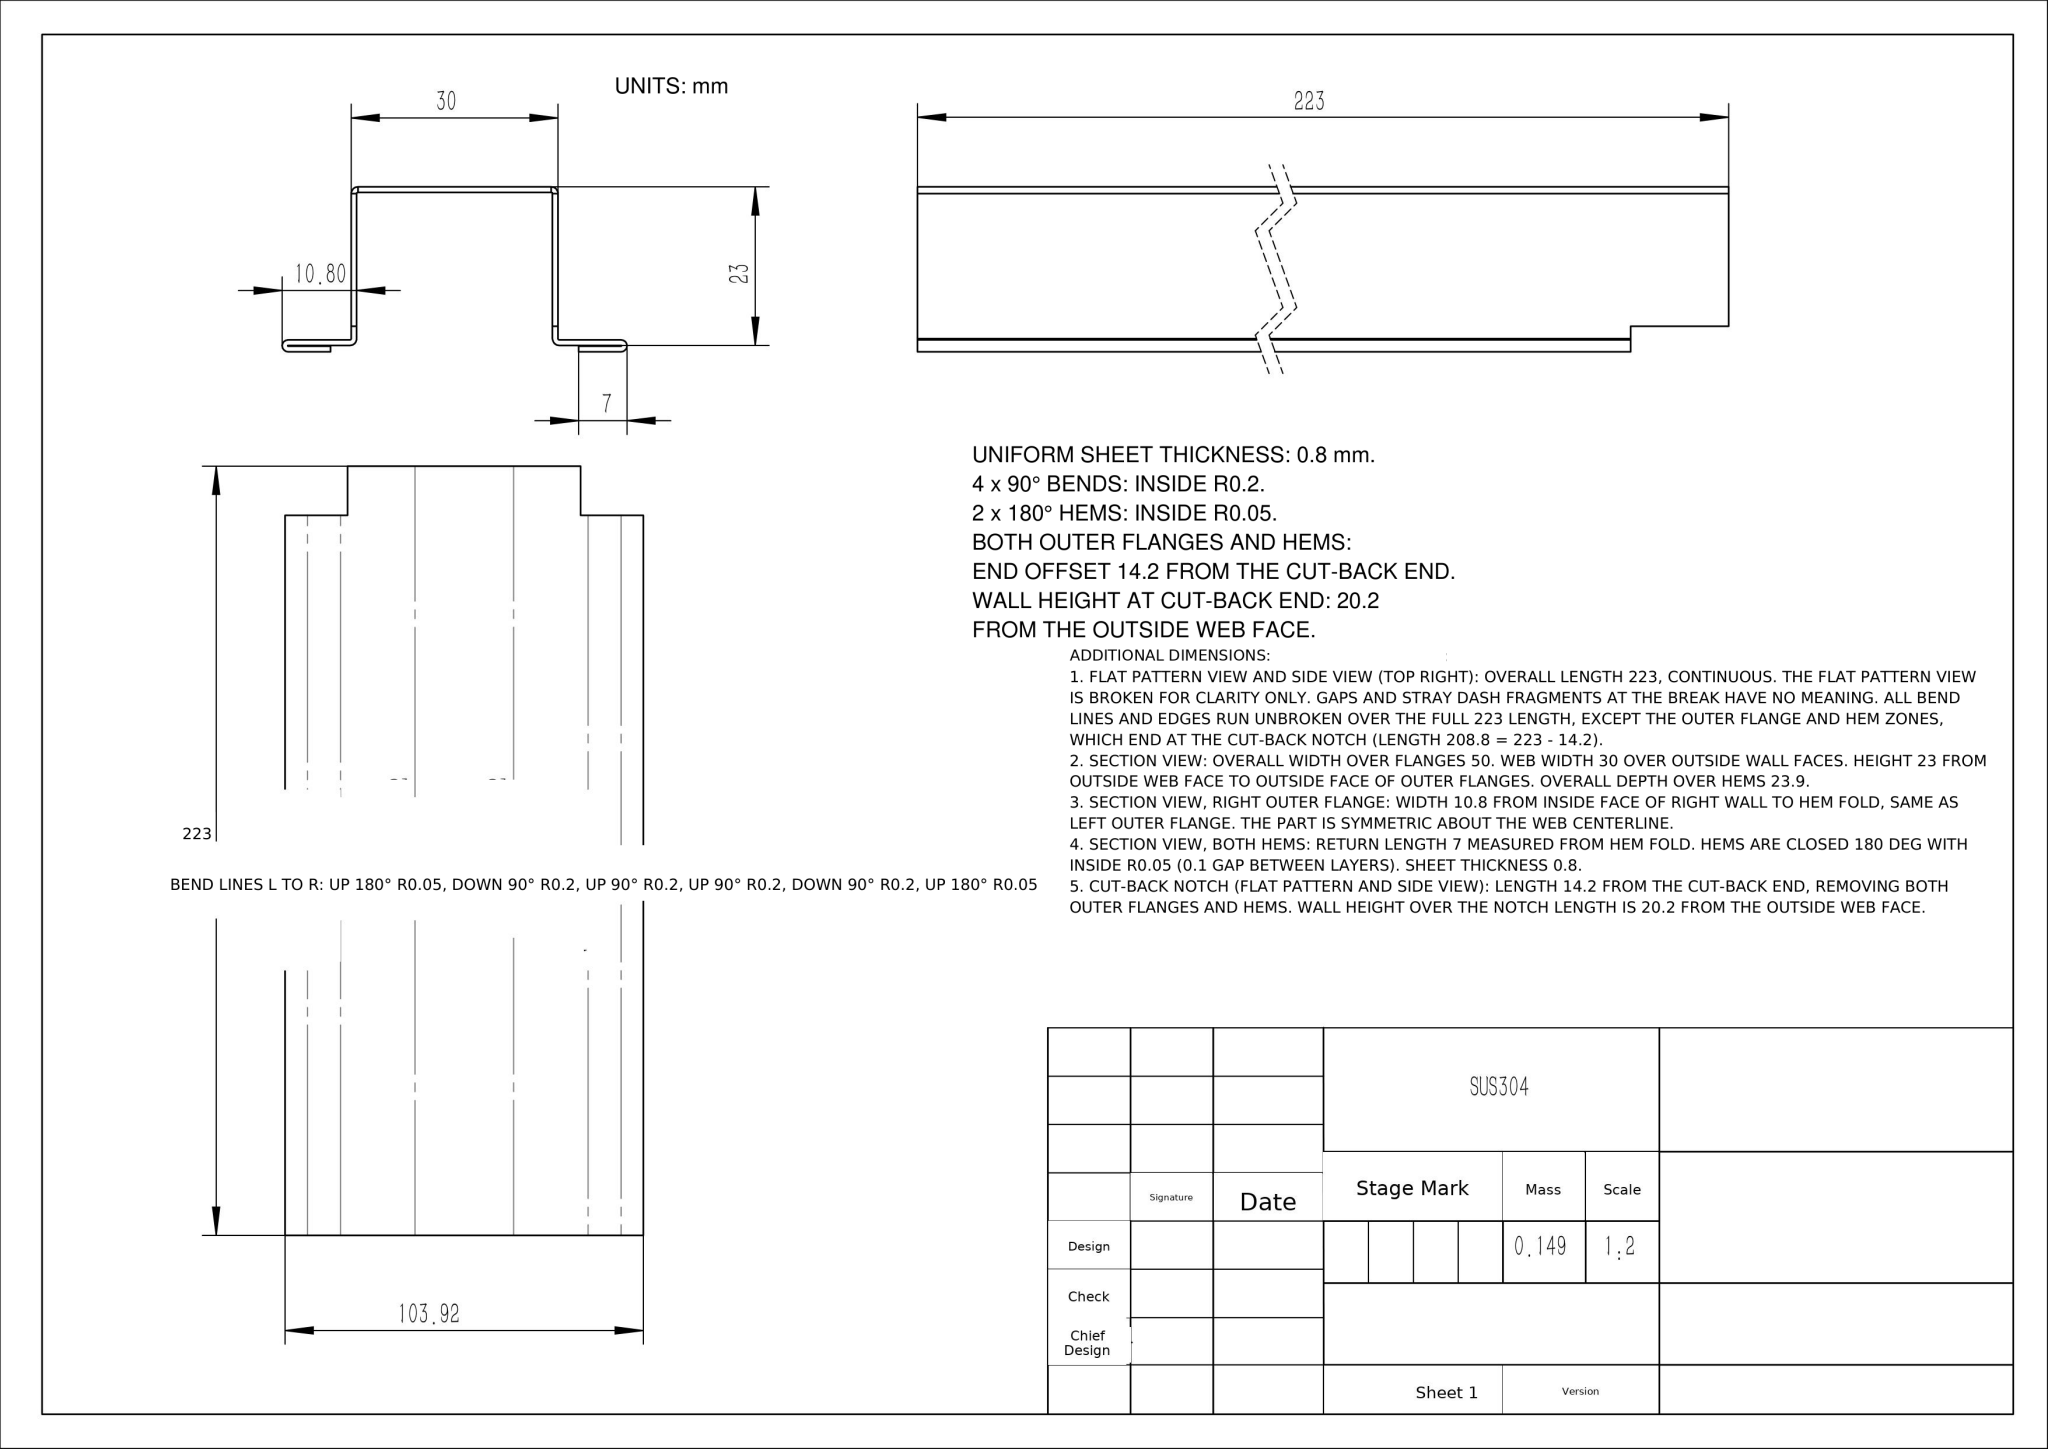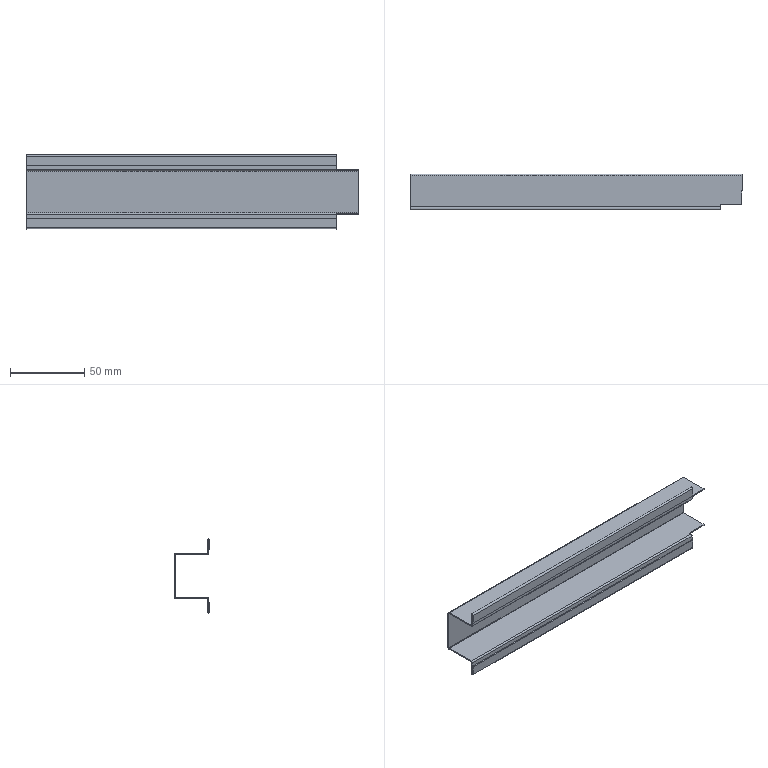Part | NX | mm | 1 solid | 50 faces | box 223 x 23.9 x 50 mm | volume 18615 mm3 | plane 38 | cylinder 12 | commonest cylinder face diameters 0.4 x4 2 x4 1.7 x2 0.1 x2